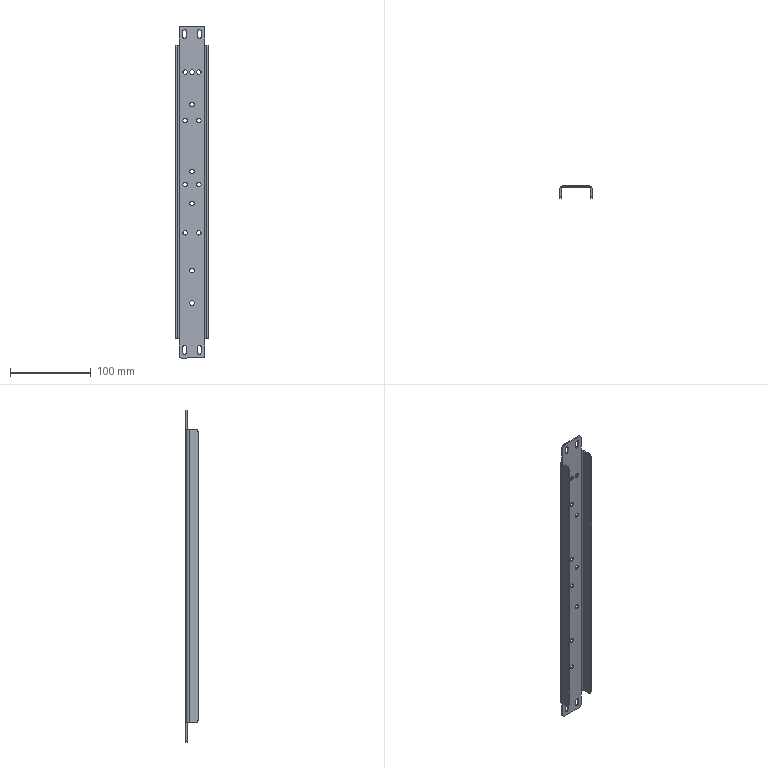Component | SolidWorks | FrameTransverseBeamTwo40001100-1 | 1 solid | 82 faces | volume 36437 mm3 | cylinder 52 | plane 30 | commonest cylinder face diameters 5.5 x40 6 x8 8 x2 5 x2